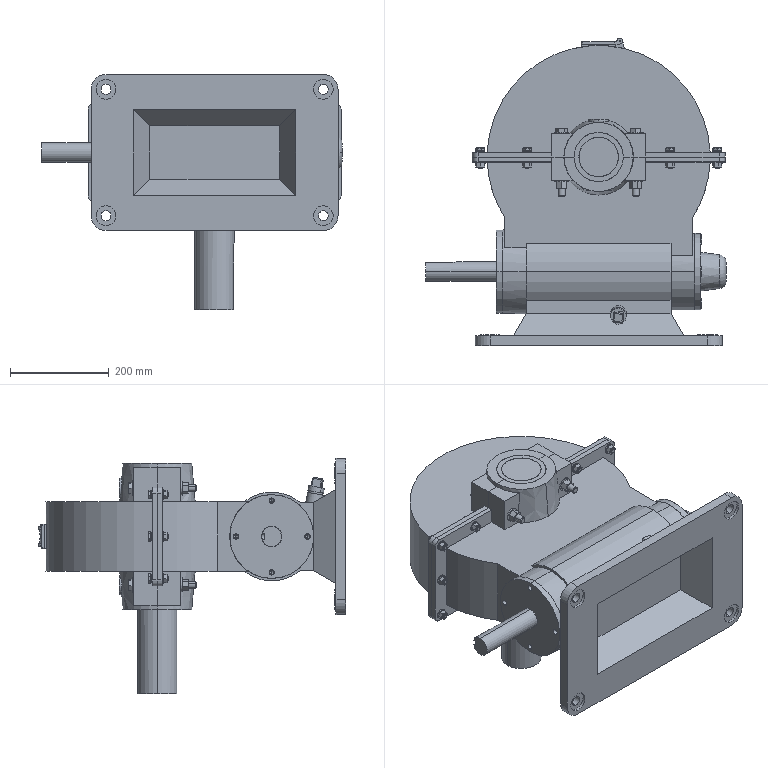Assembly | SolidWorks | mm | 63 component files | 63 solids | 1988 faces | box 608.2 x 623 x 476 mm | volume 18527930 mm3 | plane 633 | cylinder 544 | cone 521 | torus 170 | sphere 118 | spline 2 | commonest cylinder face diameters 11 x56 10 x40 16 x38 20 x36 40 x24 60 x20 100 x20 18 x20
Bill of materials:
10BearingLockPlate | 1 |  | Thin flat circular ring with a narrow rectangular cross-section; the radial width is small compared with the diameter.
11O-ring | 1 |  | Slender closed circular ring with a round cross-section, a toroidal shape.
12RearCover | 1 |  | Round flanged part: a circular flange with four evenly spaced through holes, a tapered boss with a rounded/domed end on one side, and a short cylindrical spigot with a circumferential groove on the other side.
13Type1HexNut_FinePitch_GradeAAndB[GBT6171-2000][M30_2] | 2 | Steel | Hexagonal prism with a central cylindrical through-bore; both end faces have curved chamfer edges at the hex corners. Hex-nut-like shape.
14HexHeadBolt_GradeAAndB[GBT5782-2000][M10_35_35] | 10 | Steel | Hex-head bolt-like part: a hexagonal head with a thin circular bearing collar underneath, then a plain cylindrical shank with a chamfered free end. The shank is fairly short, about 3 to 4 shank diameters long.
15FlatWasherGradeA[GBT97_1-2002][10] | 10 | Steel | Flat annular disc (washer-like) with a central round hole about half the outer diameter; its thickness is small compared with the diameter.
16Type1HexNut_GradeAAndB[GBT6170-2000][M10] | 10 | Steel | Hexagonal prism with a central cylindrical through-bore and curved chamfers on the corner edges of both end faces. Hex-nut-like shape, similar to the other hex-with-bore parts.
17WormGearShaft | 1 |  | Stepped cylindrical shaft/pin with a larger-diameter collar near one end, a small notch in the collar, and a rounded-end longitudinal slot (keyway-like) near the other end.
18Bushing | 2 |  | Thin-walled cylindrical sleeve with a narrow outward flange at each end and one small radial hole through the wall.
1CoverBox | 1 |  | Half-round (semicircular) hollow housing shell with a flat rectangular perimeter flange carrying several holes. It has two semicircular bore cutouts with surrounding bosses on opposite faces, a small rectangular opening in the center region, and a small lug on the curved outer surface.
21FuelTankCapPin | 1 |  | Long slender cylindrical pin with a domed (round) head at one end and a flat other end.
22FuelTankCap | 1 |  | Flat rectangular plate with rounded corners and two lugs projecting from one edge. Each lug has a rounded eye with a small through hole.
23HexHeadBolt_GradeAAndB[GBT5782-2000][M14_130_40] | 4 | Steel | Long, slender hex-head bolt-like part: a hexagonal head with a thin round collar underneath and a long plain cylindrical shank with a chamfered end. Length is roughly 12 to 14 shank diameters.
24FlatWasher_GradeA[GBT97_1-2002][14] | 4 | Alloy Steel | Flat annular disc (washer-like) with a central round hole about half the outer diameter; it is thin relative to the diameter.
25Type1HexNut_GradeAAndB[GBT6170-2000][M14] | 4 | Steel | Hexagonal prism with a central cylindrical through-bore; both ends have curved corner chamfers. Hex-nut-like shape, with a slightly larger thickness-to-width ratio than the other hex-with-bore parts in its own views.
26Washer | 1 |  | Flat annular ring (washer-like) with a central round hole a little over half the outer diameter. It is moderately thick relative to the diameter.
27PlugScrew | 1 |  | Stepped pin with a square block head that has chamfered edges, a larger round collar below the head, and a smaller cylindrical shank with a chamfered end.
2Housing | 1 |  | Hollow box-like housing body with a rectangular flange at each of two opposite ends, a horizontal cylindrical boss running across it, a circular side face with a central bore, and a half-round saddle (U-shaped cradle) with two square blocks on the top.
3FrontCover | 1 |  | Flanged hollow cylindrical sleeve: a thin circular flange with four through-holes, and a tubular spigot with stepped and grooved outer diameters sticking out from one side.
4OilSeal | 1 |  | Plain flat annular ring (washer- or spacer-like) with a rectangular cross-section.
5Nut | 1 |  | Thick annular ring with four rectangular notches spaced evenly around the outer edge, looking like a slotted round nut or lock ring.
6O-ring | 1 |  | Very thin circular ring with a round wire-like cross-section, looking like an O-ring or seal ring.
7DeepGrooveBallBearing276[GBT276-2013][6309] | 1 | GCr4 | Ball-bearing-like assembly: an outer ring and an inner ring with a row of spherical balls between them; no cage or shields are visible.
8Worm | 1 |  | Stepped cylindrical shaft with a helical thread section in the middle, looking like a worm shaft, with journals of different diameters on each end.
3209A | 1 | GCr4 | Rolling-element-bearing-like ring assembly: a plain cylindrical outer ring and a narrower inner ring, with about 14 spherical balls spaced evenly in the annular gap. No cage or seal is visible from the viewed face.
Mates:
1. coincident | 2Housing-1 face at (-204.115, 141.809, 612) dir (0, 0, 1) | 1CoverBox-1 face at (-204.115, 151.809, 612) dir (0, 0, 1)
2. coincident | 2Housing-1 face at (-216.115, 141.809, 424) dir (-1, 0, 0) | 1CoverBox-1 face at (-216.115, 151.809, 424) dir (-1, 0, 0)
3. coincident | 2Housing-1 face at (283.885, 141.809, 424) dir (0, 1, 0) | 1CoverBox-1 face at (283.885, 141.809, 424) dir (0, -1, 0)
4. concentric | 3FrontCover-1 face at (-162.115, -90.191, 512) dir (1, 0, 0) r 26.5 | 4OilSeal-1 face at (-156.715, -90.191, 512) dir (-1, 0, 0) r 20
5. coincident | 3FrontCover-1 face at (-156.715, -90.191, 512) dir (-1, 0, 0) | 4OilSeal-1 face at (-156.715, -90.191, 512) dir (1, 0, 0)
6. concentric | 3FrontCover-1 face at (-135.115, -90.191, 512) dir (1, 0, 0) r 58 | 6O-ring-1 axis at (-111.947, -90.191, 512) dir (-1, 0, 0)
7. tangent | 3FrontCover-1 face at (-146.89, -90.191, 512) dir (1, 0, 0) | 6O-ring-1 face at (-145.89, -90.191, 512) dir (1, 0, 0)
8. concentric | 2Housing-1 face at (-135.115, -90.191, 512) dir (-1, 0, 0) r 60 | 3FrontCover-1 axis at (-102.115, -90.191, 512) dir (-1, 0, 0)
9. coincident | 2Housing-1 axis at (-150.115, -90.191, 512) dir (1, 0, 0) | 5Nut-1 axis at (-129.115, -90.191, 512) dir (-1, 0, 0)
10. coincident | 8Worm-1 face at (-129.115, -90.191, 512) dir (1, 0, 0) | 5Nut-1 face at (-129.115, -90.191, 512) dir (1, 0, 0)
11. coincident | 8Worm-1 axis at (-145.115, -90.191, 512) dir (-1, 0, 0) | 5Nut-1 axis at (-129.115, -90.191, 512) dir (-1, 0, 0)
12. parallel | 1CoverBox-1 face at (283.885, 151.809, 424) dir (0, 1, 0) | 8Worm-1 face at (-404.295, -76.191, 512) dir (0, 1, 0)
13. concentric | 8Worm-1 face at (-213.747, -90.191, 512) dir (-1, 0, 0) r 27.5 | 7DeepGrooveBallBearing276[GBT276-2013][6309]-1 face at (-128.036, -90.191, 512) dir (-1, 0, 0) r 22.5
14. coincident | 8Worm-1 face at (-103.115, -90.191, 512) dir (-1, 0, 0) | 7DeepGrooveBallBearing276[GBT276-2013][6309]-1 face at (-103.115, -48.871, 537.394) dir (1, 0, 0)
15. concentric | 8Worm-1 face at (210.085, -90.191, 512) dir (-1, 0, 0) r 22.5 | 11O-ring-1 axis at (200.363, -90.191, 512) dir (1, 0, 0)
16. concentric | 8Worm-1 face at (210.085, -90.191, 512) dir (-1, 0, 0) r 22.5 | 12RearCover-1 axis at (311.097, -90.191, 512) dir (-1, 0, 0)
17. tangent | 11O-ring-1 face at (224.41, -90.191, 512) dir (1, 0, 0) | 12RearCover-1 face at (225.66, -90.191, 512) dir (-1, 0, 0)
18. concentric | 2Housing-1 face at (234.885, -25.191, 512) dir (1, 0, 0) r 4.25 | 12RearCover-1 face at (213.085, -25.191, 512) dir (1, 0, 0) r 5.5
19. concentric | 8Worm-1 face at (-213.747, -90.191, 512) dir (-1, 0, 0) r 27.5 | 9DoubleRowAngularContactBallBearing[GBT296-2015][3209A]-1 face at (179.885, -90.191, 512) dir (-1, 0, 0) r 22.5
20. coincident | 8Worm-1 face at (179.885, -62.691, 512) dir (1, 0, 0) | 9DoubleRowAngularContactBallBearing[GBT296-2015][3209A]-1 face at (179.885, -48.852, 521.867) dir (-1, 0, 0)
21. concentric | 8Worm-1 face at (274.085, -90.191, 512) dir (-1, 0, 0) r 15 | 13Type1HexNut_FinePitch_GradeAAndB[GBT6171-2000][M30_2]-1 face at (210.085, -90.191, 512) dir (1, 0, 0) r 15
22. coincident | 8Worm-1 axis at (274.085, -90.191, 512) dir (-1, 0, 0) | 13Type1HexNut_FinePitch_GradeAAndB[GBT6171-2000][M30_2]-2 axis at (259.164, -90.191, 512) dir (1, 0, 0)
23. coincident | 13Type1HexNut_FinePitch_GradeAAndB[GBT6171-2000][M30_2]-1 face at (235.685, -65.067, 515.903) dir (1, 0, 0) | 13Type1HexNut_FinePitch_GradeAAndB[GBT6171-2000][M30_2]-2 face at (235.685, -65.067, 515.903) dir (-1, 0, 0)
24. concentric | 8Worm-1 face at (274.085, -90.191, 512) dir (-1, 0, 0) r 15 | 10BearingLockPlate-1 face at (210.085, -90.191, 512) dir (1, 0, 0) r 39
25. coincident | 13Type1HexNut_FinePitch_GradeAAndB[GBT6171-2000][M30_2]-1 face at (210.085, -99.373, 488.291) dir (0, -0.779, -0.627) | 13Type1HexNut_FinePitch_GradeAAndB[GBT6171-2000][M30_2]-2 face at (235.685, -99.373, 488.291) dir (0, -0.779, -0.627)
26. concentric | 2Housing-1 face at (-155.115, -17.691, 512) dir (-1, 0, 0) r 4.25 | 3FrontCover-1 face at (-167.115, -17.691, 512) dir (1, 0, 0) r 5.5
27. coincident | 2Housing-1 face at (-155.115, -90.191, 512) dir (-1, 0, 0) | 3FrontCover-1 face at (-155.115, -90.191, 512) dir (1, 0, 0)
28. coincident | 2Housing-1 face at (234.885, -90.191, 512) dir (1, 0, 0) | 12RearCover-1 face at (234.885, -90.191, 469.5) dir (-1, 0, 0)
29. coincident | 8Worm-1 face at (210.085, -90.191, 512) dir (1, 0, 0) | 13Type1HexNut_FinePitch_GradeAAndB[GBT6171-2000][M30_2]-1 face at (210.085, -65.067, 515.903) dir (-1, 0, 0)
30. concentric | 2Housing-1 axis at (79.885, -175.356, 580.99) dir (0, -0.1736, 0.9848) | 26Washer-1 edge at (79.885, -179.167, 602.602) dir (0, -0.1736, 0.9848) r 8
31. concentric | 27PlugScrew-1 axis at (79.885, -176.215, 585.861) dir (0, -0.1736, 0.9848) | 26Washer-1 edge at (79.885, -179.167, 602.602) dir (0, -0.1736, 0.9848) r 8
32. coincident | 2Housing-1 face at (79.885, -178.472, 598.663) dir (0, -0.1736, 0.9848) | 26Washer-1 face at (79.885, -178.472, 598.663) dir (0, 0.1736, -0.9848)
33. coincident | 27PlugScrew-1 face at (79.885, -179.167, 602.602) dir (0, 0.1736, -0.9848) | 26Washer-1 face at (79.885, -179.167, 602.602) dir (0, -0.1736, 0.9848)
34. concentric | 2Housing-1 axis at (39.885, 141.809, 652) dir (0, 0, -1) | 17WormGearShaft-1 face at (39.885, 141.809, 194) dir (0, 0, 1) r 40
35. concentric | 1CoverBox-1 face at (82.885, 376.809, 497.5) dir (0, 0, 1) r 1.5 | 22FuelTankCap-1 axis at (82.885, 376.809, 492) dir (0, 0, 1)
36. distance | 1CoverBox-1 face at (82.885, 373.809, 526.5) dir (0, 0, 1) | 22FuelTankCap-1 face at (39.885, 370.809, 527) dir (0, 0, -1)
37. coincident | 21FuelTankCapPin-1 axis at (82.885, 376.809, 536) dir (0, 0, -1) | 22FuelTankCap-1 axis at (82.885, 376.809, 492) dir (0, 0, 1)
38. coincident | 21FuelTankCapPin-1 face at (82.885, 376.809, 492) dir (0, 0, 1) | 22FuelTankCap-1 face at (39.885, 370.809, 492) dir (0, 0, -1)
39. concentric | 2Housing-1 face at (39.885, 141.809, 372) dir (0, 0, 1) r 45 | 18Bushing-1 face at (39.885, 141.809, 464) dir (0, 0, -1) r 40
40. coincident | 1CoverBox-1 face at (39.885, 141.809, 464) dir (0, 0, 1) | 18Bushing-1 face at (39.885, 141.809, 464) dir (0, 0, 1)
41. concentric | 2Housing-1 face at (39.885, 141.809, 652) dir (0, 0, -1) r 45 | 18Bushing-2 face at (39.885, 141.809, 652) dir (0, 0, -1) r 45
42. coincident | 1CoverBox-1 face at (-30.115, 141.809, 660) dir (0, 0, 1) | 18Bushing-2 face at (39.885, 141.809, 660) dir (0, 0, 1)
43. coincident | 17WormGearShaft-1 face at (39.885, 141.809, 464) dir (0, 0, -1) | 18Bushing-1 face at (39.885, 141.809, 464) dir (0, 0, 1)
44. concentric | 1CoverBox-1 face at (-35.115, 191.809, 610) dir (0, -1, 0) r 15 | 23HexHeadBolt_GradeAAndB[GBT5782-2000][M14_130_40]-1 face at (-35.115, 200.609, 610) dir (0, 1, 0) r 7
45. coincident | 1CoverBox-1 face at (-35.115, 191.809, 610) dir (0, 1, 0) | 23HexHeadBolt_GradeAAndB[GBT5782-2000][M14_130_40]-1 face at (-29.622, 191.809, 620.808) dir (0, -1, 0)
46. concentric | 24FlatWasher_GradeA[GBT97_1-2002][14]-1 face at (-35.115, 82.664, 610) dir (0, -1, 0) r 7.5 | 23HexHeadBolt_GradeAAndB[GBT5782-2000][M14_130_40]-1 face at (-35.115, 200.609, 610) dir (0, 1, 0) r 7
47. coincident | 2Housing-1 face at (39.885, 93.809, 652) dir (0, -1, 0) | 24FlatWasher_GradeA[GBT97_1-2002][14]-1 face at (-27.91, 93.809, 612.08) dir (0, 1, 0)
48. concentric | 23HexHeadBolt_GradeAAndB[GBT5782-2000][M14_130_40]-1 face at (-35.115, 200.609, 610) dir (0, 1, 0) r 7 | 25Type1HexNut_GradeAAndB[GBT6170-2000][M14]-1 face at (-35.115, 78.509, 610) dir (0, 1, 0) r 7
49. coincident | 24FlatWasher_GradeA[GBT97_1-2002][14]-1 face at (-27.91, 91.309, 612.08) dir (0, -1, 0) | 25Type1HexNut_GradeAAndB[GBT6170-2000][M14]-1 face at (-24.715, 91.309, 604.685) dir (0, 1, 0)
50. concentric | 1CoverBox-1 face at (114.885, 141.809, 610) dir (0, 1, 0) r 8 | 23HexHeadBolt_GradeAAndB[GBT5782-2000][M14_130_40]-4 face at (114.885, 200.609, 610) dir (0, 1, 0) r 7
51. coincident | 1CoverBox-1 face at (114.885, 191.809, 610) dir (0, 1, 0) | 23HexHeadBolt_GradeAAndB[GBT5782-2000][M14_130_40]-4 face at (114.664, 191.809, 622.122) dir (0, -1, 0)
52. concentric | 1CoverBox-1 face at (114.885, 141.809, 414) dir (0, 1, 0) r 8 | 23HexHeadBolt_GradeAAndB[GBT5782-2000][M14_130_40]-5 face at (114.885, 200.609, 414) dir (0, 1, 0) r 7
53. coincident | 1CoverBox-1 face at (114.885, 191.809, 414) dir (0, 1, 0) | 23HexHeadBolt_GradeAAndB[GBT5782-2000][M14_130_40]-5 face at (116.953, 191.809, 425.947) dir (0, -1, 0)
54. concentric | 1CoverBox-1 face at (-35.115, 141.809, 414) dir (0, 1, 0) r 8 | 23HexHeadBolt_GradeAAndB[GBT5782-2000][M14_130_40]-7 face at (-35.115, 200.609, 414) dir (0, 1, 0) r 7
55. coincident | 1CoverBox-1 face at (-35.115, 191.809, 414) dir (0, 1, 0) | 23HexHeadBolt_GradeAAndB[GBT5782-2000][M14_130_40]-7 face at (-30.52, 191.809, 425.22) dir (0, -1, 0)
56. concentric | 23HexHeadBolt_GradeAAndB[GBT5782-2000][M14_130_40]-4 face at (114.885, 200.609, 610) dir (0, 1, 0) r 7 | 24FlatWasher_GradeA[GBT97_1-2002][14]-2 face at (114.885, 82.664, 610) dir (0, -1, 0) r 14
57. coincident | 2Housing-1 face at (39.885, 93.809, 652) dir (0, -1, 0) | 24FlatWasher_GradeA[GBT97_1-2002][14]-2 face at (107.385, 93.809, 610) dir (0, 1, 0)
58. concentric | 23HexHeadBolt_GradeAAndB[GBT5782-2000][M14_130_40]-5 face at (114.885, 200.609, 414) dir (0, 1, 0) r 7 | 24FlatWasher_GradeA[GBT97_1-2002][14]-3 face at (114.885, 82.664, 414) dir (0, -1, 0) r 14
59. coincident | 2Housing-1 face at (39.885, 93.809, 372) dir (0, -1, 0) | 24FlatWasher_GradeA[GBT97_1-2002][14]-3 face at (107.519, 93.809, 415.413) dir (0, 1, 0)
60. concentric | 23HexHeadBolt_GradeAAndB[GBT5782-2000][M14_130_40]-7 face at (-35.115, 200.609, 414) dir (0, 1, 0) r 7 | 24FlatWasher_GradeA[GBT97_1-2002][14]-5 face at (-35.115, 82.664, 414) dir (0, -1, 0) r 14
61. coincident | 2Housing-1 face at (39.885, 93.809, 372) dir (0, -1, 0) | 24FlatWasher_GradeA[GBT97_1-2002][14]-5 face at (-42.003, 93.809, 416.968) dir (0, 1, 0)
62. concentric | 23HexHeadBolt_GradeAAndB[GBT5782-2000][M14_130_40]-5 axis at (114.885, 63.409, 414) dir (0, 1, 0) | 25Type1HexNut_GradeAAndB[GBT6170-2000][M14]-2 edge at (114.885, 79.392, 414) dir (0, -1, 0) r 7
63. coincident | 24FlatWasher_GradeA[GBT97_1-2002][14]-3 face at (107.519, 91.309, 415.413) dir (0, -1, 0) | 25Type1HexNut_GradeAAndB[GBT6170-2000][M14]-2 face at (125.023, 91.309, 408.2) dir (0, 1, 0)
64. concentric | 23HexHeadBolt_GradeAAndB[GBT5782-2000][M14_130_40]-7 face at (-35.115, 200.609, 414) dir (0, 1, 0) r 7 | 25Type1HexNut_GradeAAndB[GBT6170-2000][M14]-3 edge at (-35.115, 79.392, 414) dir (0, -1, 0) r 7
65. coincident | 24FlatWasher_GradeA[GBT97_1-2002][14]-5 face at (-42.003, 91.309, 416.968) dir (0, -1, 0) | 25Type1HexNut_GradeAAndB[GBT6170-2000][M14]-3 face at (-26.252, 91.309, 406.393) dir (0, 1, 0)
66. concentric | 23HexHeadBolt_GradeAAndB[GBT5782-2000][M14_130_40]-4 axis at (114.885, 63.409, 610) dir (0, 1, 0) | 25Type1HexNut_GradeAAndB[GBT6170-2000][M14]-5 edge at (114.885, 79.392, 610) dir (0, -1, 0) r 7
67. coincident | 24FlatWasher_GradeA[GBT97_1-2002][14]-2 face at (107.385, 91.309, 610) dir (0, -1, 0) | 25Type1HexNut_GradeAAndB[GBT6170-2000][M14]-5 face at (121.9, 91.309, 600.661) dir (0, 1, 0)
68. concentric | 1CoverBox-1 face at (-200.115, 141.809, 427) dir (0, 1, 0) r 5.5 | 14HexHeadBolt_GradeAAndB[GBT5782-2000][M10_35_35]-1 axis at (-200.115, 120.009, 427) dir (0, 1, 0)
69. coincident | 1CoverBox-1 face at (-200.115, 153.809, 427) dir (0, 1, 0) | 14HexHeadBolt_GradeAAndB[GBT5782-2000][M10_35_35]-1 face at (-192.382, 153.809, 432.052) dir (0, -1, 0)
70. concentric | 1CoverBox-1 face at (-200.115, 141.809, 512) dir (0, 1, 0) r 5.5 | 14HexHeadBolt_GradeAAndB[GBT5782-2000][M10_35_35]-3 axis at (-200.115, 120.009, 512) dir (0, 1, 0)
71. coincident | 1CoverBox-1 face at (-200.115, 153.809, 512) dir (0, 1, 0) | 14HexHeadBolt_GradeAAndB[GBT5782-2000][M10_35_35]-3 face at (-191.568, 153.809, 515.505) dir (0, -1, 0)
72. concentric | 1CoverBox-1 face at (-200.115, 141.809, 597) dir (0, 1, 0) r 5.5 | 14HexHeadBolt_GradeAAndB[GBT5782-2000][M10_35_35]-5 axis at (-200.115, 120.009, 597) dir (0, 1, 0)
73. coincident | 1CoverBox-1 face at (-200.115, 153.809, 597) dir (0, 1, 0) | 14HexHeadBolt_GradeAAndB[GBT5782-2000][M10_35_35]-5 face at (-191.014, 153.809, 598.58) dir (0, -1, 0)
74. concentric | 1CoverBox-1 face at (-105.115, 141.809, 597) dir (0, 1, 0) r 5.5 | 14HexHeadBolt_GradeAAndB[GBT5782-2000][M10_35_35]-7 axis at (-105.115, 120.009, 597) dir (0, 1, 0)
75. coincident | 1CoverBox-1 face at (-105.115, 153.809, 597) dir (0, 1, 0) | 14HexHeadBolt_GradeAAndB[GBT5782-2000][M10_35_35]-7 face at (-95.897, 153.809, 596.402) dir (0, -1, 0)
76. concentric | 1CoverBox-1 face at (184.885, 141.809, 597) dir (0, 1, 0) r 5.5 | 14HexHeadBolt_GradeAAndB[GBT5782-2000][M10_35_35]-9 axis at (184.885, 120.009, 597) dir (0, 1, 0)
77. coincident | 1CoverBox-1 face at (184.885, 153.809, 597) dir (0, 1, 0) | 14HexHeadBolt_GradeAAndB[GBT5782-2000][M10_35_35]-9 face at (193.693, 153.809, 594.218) dir (0, -1, 0)
78. concentric | 1CoverBox-1 face at (279.885, 141.809, 597) dir (0, 1, 0) r 5.5 | 14HexHeadBolt_GradeAAndB[GBT5782-2000][M10_35_35]-11 axis at (279.885, 120.009, 597) dir (0, 1, 0)
79. coincident | 1CoverBox-1 face at (279.885, 153.809, 597) dir (0, 1, 0) | 14HexHeadBolt_GradeAAndB[GBT5782-2000][M10_35_35]-11 face at (287.843, 153.809, 592.311) dir (0, -1, 0)
80. concentric | 1CoverBox-1 face at (279.885, 141.809, 512) dir (0, 1, 0) r 5.5 | 14HexHeadBolt_GradeAAndB[GBT5782-2000][M10_35_35]-13 axis at (279.885, 120.009, 512) dir (0, 1, 0)
81. coincident | 1CoverBox-1 face at (279.885, 153.809, 512) dir (0, 1, 0) | 14HexHeadBolt_GradeAAndB[GBT5782-2000][M10_35_35]-13 face at (286.795, 153.809, 505.869) dir (0, -1, 0)
82. concentric | 1CoverBox-1 face at (279.885, 141.809, 427) dir (0, 1, 0) r 5.5 | 14HexHeadBolt_GradeAAndB[GBT5782-2000][M10_35_35]-15 axis at (279.885, 120.009, 427) dir (0, 1, 0)
83. coincident | 1CoverBox-1 face at (279.885, 153.809, 427) dir (0, 1, 0) | 14HexHeadBolt_GradeAAndB[GBT5782-2000][M10_35_35]-15 face at (285.83, 153.809, 419.93) dir (0, -1, 0)
84. concentric | 1CoverBox-1 face at (184.885, 141.809, 427) dir (0, 1, 0) r 5.5 | 14HexHeadBolt_GradeAAndB[GBT5782-2000][M10_35_35]-17 axis at (184.885, 120.009, 427) dir (0, 1, 0)
85. coincident | 1CoverBox-1 face at (184.885, 153.809, 427) dir (0, 1, 0) | 14HexHeadBolt_GradeAAndB[GBT5782-2000][M10_35_35]-17 face at (190.17, 153.809, 419.424) dir (0, -1, 0)
86. concentric | 1CoverBox-1 face at (-105.115, 141.809, 427) dir (0, 1, 0) r 5.5 | 14HexHeadBolt_GradeAAndB[GBT5782-2000][M10_35_35]-20 axis at (-105.115, 120.009, 427) dir (0, 1, 0)
87. coincident | 1CoverBox-1 face at (-105.115, 153.809, 427) dir (0, 1, 0) | 14HexHeadBolt_GradeAAndB[GBT5782-2000][M10_35_35]-20 face at (-100.063, 153.809, 419.267) dir (0, -1, 0)
88. concentric | 14HexHeadBolt_GradeAAndB[GBT5782-2000][M10_35_35]-1 face at (-200.115, 160.209, 427) dir (0, 1, 0) r 5 | 15FlatWasherGradeA[GBT97_1-2002][10]-2 face at (-200.115, 131.809, 427) dir (0, -1, 0) r 5.25
89. coincident | 2Housing-1 face at (283.885, 131.809, 424) dir (0, -1, 0) | 15FlatWasherGradeA[GBT97_1-2002][10]-2 face at (-200.115, 131.809, 427) dir (0, 1, 0)
90. concentric | 14HexHeadBolt_GradeAAndB[GBT5782-2000][M10_35_35]-3 face at (-200.115, 160.209, 512) dir (0, 1, 0) r 5 | 15FlatWasherGradeA[GBT97_1-2002][10]-3 face at (-200.115, 131.809, 512) dir (0, -1, 0) r 5.25
91. coincident | 2Housing-1 face at (283.885, 131.809, 424) dir (0, -1, 0) | 15FlatWasherGradeA[GBT97_1-2002][10]-3 face at (-200.115, 131.809, 512) dir (0, 1, 0)
92. concentric | 14HexHeadBolt_GradeAAndB[GBT5782-2000][M10_35_35]-5 face at (-200.115, 160.209, 597) dir (0, 1, 0) r 5 | 15FlatWasherGradeA[GBT97_1-2002][10]-5 face at (-200.115, 131.809, 597) dir (0, -1, 0) r 5.25
93. coincident | 2Housing-1 face at (283.885, 131.809, 424) dir (0, -1, 0) | 15FlatWasherGradeA[GBT97_1-2002][10]-5 face at (-200.115, 131.809, 597) dir (0, 1, 0)
94. concentric | 14HexHeadBolt_GradeAAndB[GBT5782-2000][M10_35_35]-7 face at (-105.115, 160.209, 597) dir (0, 1, 0) r 5 | 15FlatWasherGradeA[GBT97_1-2002][10]-7 face at (-105.115, 131.809, 597) dir (0, -1, 0) r 5.25
95. coincident | 2Housing-1 face at (283.885, 131.809, 424) dir (0, -1, 0) | 15FlatWasherGradeA[GBT97_1-2002][10]-7 face at (-105.115, 131.809, 597) dir (0, 1, 0)
96. concentric | 14HexHeadBolt_GradeAAndB[GBT5782-2000][M10_35_35]-9 face at (184.885, 160.209, 597) dir (0, 1, 0) r 5 | 15FlatWasherGradeA[GBT97_1-2002][10]-9 face at (184.885, 131.809, 597) dir (0, -1, 0) r 5.25
97. coincident | 2Housing-1 face at (283.885, 131.809, 424) dir (0, -1, 0) | 15FlatWasherGradeA[GBT97_1-2002][10]-9 face at (184.885, 131.809, 597) dir (0, 1, 0)
98. concentric | 14HexHeadBolt_GradeAAndB[GBT5782-2000][M10_35_35]-11 face at (279.885, 160.209, 597) dir (0, 1, 0) r 5 | 15FlatWasherGradeA[GBT97_1-2002][10]-11 face at (279.885, 131.809, 597) dir (0, -1, 0) r 5.25
99. coincident | 2Housing-1 face at (283.885, 131.809, 424) dir (0, -1, 0) | 15FlatWasherGradeA[GBT97_1-2002][10]-11 face at (279.885, 131.809, 597) dir (0, 1, 0)
100. concentric | 14HexHeadBolt_GradeAAndB[GBT5782-2000][M10_35_35]-13 face at (279.885, 160.209, 512) dir (0, 1, 0) r 5 | 15FlatWasherGradeA[GBT97_1-2002][10]-13 face at (279.885, 131.809, 512) dir (0, -1, 0) r 5.25
101. coincident | 2Housing-1 face at (283.885, 131.809, 424) dir (0, -1, 0) | 15FlatWasherGradeA[GBT97_1-2002][10]-13 face at (279.885, 131.809, 512) dir (0, 1, 0)
102. concentric | 14HexHeadBolt_GradeAAndB[GBT5782-2000][M10_35_35]-15 face at (279.885, 160.209, 427) dir (0, 1, 0) r 5 | 15FlatWasherGradeA[GBT97_1-2002][10]-16 face at (279.885, 131.809, 427) dir (0, -1, 0) r 5.25
103. coincident | 2Housing-1 face at (283.885, 131.809, 424) dir (0, -1, 0) | 15FlatWasherGradeA[GBT97_1-2002][10]-16 face at (279.885, 131.809, 427) dir (0, 1, 0)
104. concentric | 14HexHeadBolt_GradeAAndB[GBT5782-2000][M10_35_35]-17 face at (184.885, 160.209, 427) dir (0, 1, 0) r 5 | 15FlatWasherGradeA[GBT97_1-2002][10]-18 face at (184.885, 131.809, 427) dir (0, -1, 0) r 5.25
105. coincident | 2Housing-1 face at (283.885, 131.809, 424) dir (0, -1, 0) | 15FlatWasherGradeA[GBT97_1-2002][10]-18 face at (184.885, 131.809, 427) dir (0, 1, 0)
106. concentric | 14HexHeadBolt_GradeAAndB[GBT5782-2000][M10_35_35]-20 face at (-105.115, 160.209, 427) dir (0, 1, 0) r 5 | 15FlatWasherGradeA[GBT97_1-2002][10]-20 face at (-105.115, 131.809, 427) dir (0, -1, 0) r 5.25
107. coincident | 2Housing-1 face at (283.885, 131.809, 424) dir (0, -1, 0) | 15FlatWasherGradeA[GBT97_1-2002][10]-20 face at (-105.115, 131.809, 427) dir (0, 1, 0)
108. concentric | 16Type1HexNut_GradeAAndB[GBT6170-2000][M10]-1 face at (-200.115, 129.809, 512) dir (0, -1, 0) r 5 | 14HexHeadBolt_GradeAAndB[GBT5782-2000][M10_35_35]-3 face at (-200.115, 160.209, 512) dir (0, 1, 0) r 5
109. coincident | 16Type1HexNut_GradeAAndB[GBT6170-2000][M10]-1 face at (-192.403, 129.809, 507.588) dir (0, 1, 0) | 15FlatWasherGradeA[GBT97_1-2002][10]-3 face at (-200.115, 129.809, 512) dir (0, -1, 0)
110. concentric | 14HexHeadBolt_GradeAAndB[GBT5782-2000][M10_35_35]-5 face at (-200.115, 160.209, 597) dir (0, 1, 0) r 5 | 16Type1HexNut_GradeAAndB[GBT6170-2000][M10]-2 face at (-200.115, 129.809, 597) dir (0, -1, 0) r 5
111. coincident | 15FlatWasherGradeA[GBT97_1-2002][10]-5 face at (-200.115, 129.809, 597) dir (0, -1, 0) | 16Type1HexNut_GradeAAndB[GBT6170-2000][M10]-2 face at (-193.373, 129.809, 591.213) dir (0, 1, 0)
112. concentric | 14HexHeadBolt_GradeAAndB[GBT5782-2000][M10_35_35]-1 face at (-200.115, 160.209, 427) dir (0, 1, 0) r 5 | 16Type1HexNut_GradeAAndB[GBT6170-2000][M10]-4 face at (-200.115, 129.809, 427) dir (0, -1, 0) r 5
113. coincident | 15FlatWasherGradeA[GBT97_1-2002][10]-2 face at (-200.115, 129.809, 427) dir (0, -1, 0) | 16Type1HexNut_GradeAAndB[GBT6170-2000][M10]-4 face at (-194.779, 129.809, 419.896) dir (0, 1, 0)
114. concentric | 14HexHeadBolt_GradeAAndB[GBT5782-2000][M10_35_35]-20 face at (-105.115, 160.209, 427) dir (0, 1, 0) r 5 | 16Type1HexNut_GradeAAndB[GBT6170-2000][M10]-6 face at (-105.115, 129.809, 427) dir (0, -1, 0) r 5
115. coincident | 15FlatWasherGradeA[GBT97_1-2002][10]-20 face at (-105.115, 129.809, 427) dir (0, -1, 0) | 16Type1HexNut_GradeAAndB[GBT6170-2000][M10]-6 face at (-101.593, 129.809, 418.843) dir (0, 1, 0)
116. concentric | 14HexHeadBolt_GradeAAndB[GBT5782-2000][M10_35_35]-17 face at (184.885, 160.209, 427) dir (0, 1, 0) r 5 | 16Type1HexNut_GradeAAndB[GBT6170-2000][M10]-8 face at (184.885, 129.809, 427) dir (0, -1, 0) r 5
117. coincident | 15FlatWasherGradeA[GBT97_1-2002][10]-18 face at (184.885, 129.809, 427) dir (0, -1, 0) | 16Type1HexNut_GradeAAndB[GBT6170-2000][M10]-8 face at (186.357, 129.809, 418.238) dir (0, 1, 0)
118. concentric | 14HexHeadBolt_GradeAAndB[GBT5782-2000][M10_35_35]-15 face at (279.885, 160.209, 427) dir (0, 1, 0) r 5 | 16Type1HexNut_GradeAAndB[GBT6170-2000][M10]-10 face at (279.885, 129.809, 427) dir (0, -1, 0) r 5
119. coincident | 15FlatWasherGradeA[GBT97_1-2002][10]-16 face at (279.885, 129.809, 427) dir (0, -1, 0) | 16Type1HexNut_GradeAAndB[GBT6170-2000][M10]-10 face at (279.352, 129.809, 418.131) dir (0, 1, 0)
120. concentric | 14HexHeadBolt_GradeAAndB[GBT5782-2000][M10_35_35]-13 face at (279.885, 160.209, 512) dir (0, 1, 0) r 5 | 16Type1HexNut_GradeAAndB[GBT6170-2000][M10]-12 face at (279.885, 129.809, 512) dir (0, -1, 0) r 5
121. coincident | 15FlatWasherGradeA[GBT97_1-2002][10]-13 face at (279.885, 129.809, 512) dir (0, -1, 0) | 16Type1HexNut_GradeAAndB[GBT6170-2000][M10]-12 face at (277.658, 129.809, 503.399) dir (0, 1, 0)
122. concentric | 14HexHeadBolt_GradeAAndB[GBT5782-2000][M10_35_35]-11 face at (279.885, 160.209, 597) dir (0, 1, 0) r 5 | 16Type1HexNut_GradeAAndB[GBT6170-2000][M10]-14 face at (279.885, 129.809, 597) dir (0, -1, 0) r 5
123. coincident | 15FlatWasherGradeA[GBT97_1-2002][10]-11 face at (279.885, 129.809, 597) dir (0, -1, 0) | 16Type1HexNut_GradeAAndB[GBT6170-2000][M10]-14 face at (276.431, 129.809, 588.814) dir (0, 1, 0)
124. concentric | 14HexHeadBolt_GradeAAndB[GBT5782-2000][M10_35_35]-9 face at (184.885, 160.209, 597) dir (0, 1, 0) r 5 | 16Type1HexNut_GradeAAndB[GBT6170-2000][M10]-16 face at (184.885, 129.809, 597) dir (0, -1, 0) r 5
125. coincident | 15FlatWasherGradeA[GBT97_1-2002][10]-9 face at (184.885, 129.809, 597) dir (0, -1, 0) | 16Type1HexNut_GradeAAndB[GBT6170-2000][M10]-16 face at (180.709, 129.809, 589.157) dir (0, 1, 0)
126. concentric | 14HexHeadBolt_GradeAAndB[GBT5782-2000][M10_35_35]-7 face at (-105.115, 160.209, 597) dir (0, 1, 0) r 5 | 16Type1HexNut_GradeAAndB[GBT6170-2000][M10]-18 face at (-105.115, 129.809, 597) dir (0, -1, 0) r 5
127. coincident | 15FlatWasherGradeA[GBT97_1-2002][10]-7 face at (-105.115, 129.809, 597) dir (0, -1, 0) | 16Type1HexNut_GradeAAndB[GBT6170-2000][M10]-18 face at (-109.528, 129.809, 589.288) dir (0, 1, 0)
128. coincident | 9DoubleRowAngularContactBallBearing[GBT296-2015][3209A]-1 face at (210.085, -48.852, 521.867) dir (1, 0, 0) | 10BearingLockPlate-1 face at (210.085, -90.191, 512) dir (-1, 0, 0)
129. coincident | 2Housing-1 face at (179.885, -90.191, 512) dir (1, 0, 0) | 9DoubleRowAngularContactBallBearing[GBT296-2015][3209A]-1 face at (179.885, -48.852, 521.867) dir (-1, 0, 0)